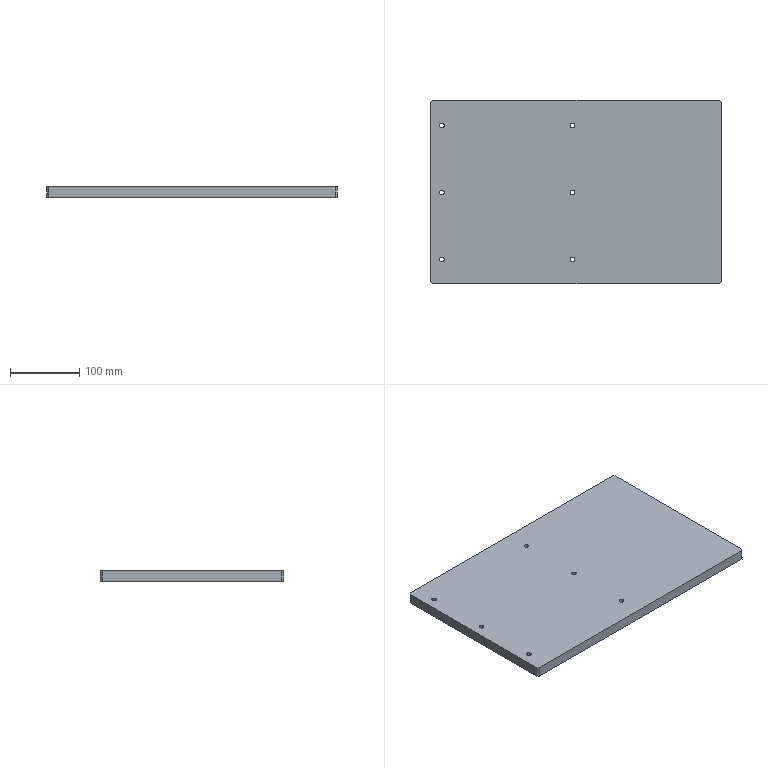Component | SolidWorks | STE21014.01-48-1 | 1 solid | 22 faces | box 420 x 265 x 15 mm | volume 1665961 mm3 | cylinder 12 | plane 10 | commonest cylinder face diameters 6.8 x12 | material Q235
build123d program:
from build123d import *

# Parameters (mm, degrees)
SKETCH1_W           = 420
SKETCH1_H           = 265
BOSS_EXTRUDE1_DEPTH = 15
M8_TAPPED_HOLE1_D   = 6.8
CHAMFER1_SIZE       = 3


with BuildPart() as part:
    # Sketch1 → Boss-Extrude1 (new body)
    with BuildSketch(Plane(origin=(0, 0, 0), x_dir=(1, 0, 0), z_dir=(0, 1, 0))):
        Rectangle(SKETCH1_W, SKETCH1_H)
    extrude(amount=BOSS_EXTRUDE1_DEPTH)

    # M8 Tapped Hole1 (through all)
    with Locations(Plane(origin=(0, 15, 0), x_dir=(1, 0, 0), z_dir=(0, 1, 0))):
        with Locations((5, -96.25), (194, -96.25), (5, 97.75), (194, 97.75), (5, 0.75), (194, 0.75)):
            Hole(M8_TAPPED_HOLE1_D / 2)

    # Chamfer1
    chamfer1_edges = [part.edges().sort_by_distance(p)[0] for p in [
        (-210, 7.5, -132.5),
        (210, 7.5, -132.5),
        (210, 7.5, 132.5),
        (-210, 7.5, 132.5),
    ]]
    chamfer(chamfer1_edges, length=CHAMFER1_SIZE)


solid = part.part

# Placed as in the assembly
solid = solid.moved(Location((530, 687.5, -105), (-90, 0, 180)))
STEP:
#1=COLOUR_RGB('',0.7922,0.8196,0.9333);
#2=FILL_AREA_STYLE_COLOUR('',#1);
#3=FILL_AREA_STYLE('',(#2));
#4=SURFACE_STYLE_FILL_AREA(#3);
#5=SURFACE_SIDE_STYLE('',(#4));
#6=SURFACE_STYLE_USAGE(.BOTH.,#5);
#7=PRESENTATION_STYLE_ASSIGNMENT((#6));
#8=CARTESIAN_POINT('',(20.669,30.722,-4.134));
#9=VERTEX_POINT('',#8);
#10=CARTESIAN_POINT('',(20.669,30.99,-4.134));
#11=VERTEX_POINT('',#10);
#12=CARTESIAN_POINT('',(20.669,30.856,-4.134));
#13=DIRECTION('',(0.,0.,1.));
#14=DIRECTION('',(0.,1.,0.));
#15=AXIS2_PLACEMENT_3D('',#12,#13,#14);
#16=CIRCLE('',#15,0.1339);
#17=EDGE_CURVE('',#9,#11,#16,.T.);
#18=ORIENTED_EDGE('',*,*,#17,.F.);
#19=CARTESIAN_POINT('',(20.669,30.722,-3.543));
#20=VERTEX_POINT('',#19);
#21=CARTESIAN_POINT('',(20.669,30.722,-3.543));
#22=DIRECTION('',(0.,0.,1.));
#23=VECTOR('',#22,39.37);
#24=LINE('',#21,#23);
#25=EDGE_CURVE('',#9,#20,#24,.T.);
#26=ORIENTED_EDGE('',*,*,#25,.T.);
#27=CARTESIAN_POINT('',(20.669,30.99,-3.543));
#28=VERTEX_POINT('',#27);
#29=CARTESIAN_POINT('',(20.669,30.856,-3.543));
#30=DIRECTION('',(0.,0.,1.));
#31=DIRECTION('',(0.,1.,0.));
#32=AXIS2_PLACEMENT_3D('',#29,#30,#31);
#33=CIRCLE('',#32,0.1339);
#34=EDGE_CURVE('',#20,#28,#33,.T.);
#35=ORIENTED_EDGE('',*,*,#34,.T.);
#36=CARTESIAN_POINT('',(20.669,30.99,-3.543));
#37=DIRECTION('',(0.,0.,1.));
#38=VECTOR('',#37,39.37);
#39=LINE('',#36,#38);
#40=EDGE_CURVE('',#11,#28,#39,.T.);
#41=ORIENTED_EDGE('',*,*,#40,.F.);
#42=EDGE_LOOP('',(#18,#26,#35,#41));
#43=FACE_OUTER_BOUND('',#42,.T.);
#44=CARTESIAN_POINT('',(20.669,30.856,-3.543));
#45=DIRECTION('',(0.,0.,1.));
#46=DIRECTION('',(0.,1.,0.));
#47=AXIS2_PLACEMENT_3D('',#44,#45,#46);
#48=CYLINDRICAL_SURFACE('',#47,0.1339);
#49=ADVANCED_FACE('',(#43),#48,.F.);
#50=CARTESIAN_POINT('',(13.228,30.722,-4.134));
#51=VERTEX_POINT('',#50);
#52=CARTESIAN_POINT('',(13.228,30.99,-4.134));
#53=VERTEX_POINT('',#52);
#54=CARTESIAN_POINT('',(13.228,30.856,-4.134));
#55=DIRECTION('',(0.,0.,1.));
#56=DIRECTION('',(0.,1.,0.));
#57=AXIS2_PLACEMENT_3D('',#54,#55,#56);
#58=CIRCLE('',#57,0.1339);
#59=EDGE_CURVE('',#51,#53,#58,.T.);
#60=ORIENTED_EDGE('',*,*,#59,.F.);
#61=CARTESIAN_POINT('',(13.228,30.722,-3.543));
#62=VERTEX_POINT('',#61);
#63=CARTESIAN_POINT('',(13.228,30.722,-3.543));
#64=DIRECTION('',(0.,0.,1.));
#65=VECTOR('',#64,39.37);
#66=LINE('',#63,#65);
#67=EDGE_CURVE('',#51,#62,#66,.T.);
#68=ORIENTED_EDGE('',*,*,#67,.T.);
#69=CARTESIAN_POINT('',(13.228,30.99,-3.543));
#70=VERTEX_POINT('',#69);
#71=CARTESIAN_POINT('',(13.228,30.856,-3.543));
#72=DIRECTION('',(0.,0.,1.));
#73=DIRECTION('',(0.,1.,0.));
#74=AXIS2_PLACEMENT_3D('',#71,#72,#73);
#75=CIRCLE('',#74,0.1339);
#76=EDGE_CURVE('',#62,#70,#75,.T.);
#77=ORIENTED_EDGE('',*,*,#76,.T.);
#78=CARTESIAN_POINT('',(13.228,30.99,-3.543));
#79=DIRECTION('',(0.,0.,1.));
#80=VECTOR('',#79,39.37);
#81=LINE('',#78,#80);
#82=EDGE_CURVE('',#53,#70,#81,.T.);
#83=ORIENTED_EDGE('',*,*,#82,.F.);
#84=EDGE_LOOP('',(#60,#68,#77,#83));
#85=FACE_OUTER_BOUND('',#84,.T.);
#86=CARTESIAN_POINT('',(13.228,30.856,-3.543));
#87=DIRECTION('',(0.,0.,1.));
#88=DIRECTION('',(0.,1.,0.));
#89=AXIS2_PLACEMENT_3D('',#86,#87,#88);
#90=CYLINDRICAL_SURFACE('',#89,0.1339);
#91=ADVANCED_FACE('',(#85),#90,.F.);
#92=CARTESIAN_POINT('',(20.669,23.085,-4.134));
#93=VERTEX_POINT('',#92);
#94=CARTESIAN_POINT('',(20.669,23.352,-4.134));
#95=VERTEX_POINT('',#94);
#96=CARTESIAN_POINT('',(20.669,23.219,-4.134));
#97=DIRECTION('',(0.,0.,1.));
#98=DIRECTION('',(0.,1.,0.));
#99=AXIS2_PLACEMENT_3D('',#96,#97,#98);
#100=CIRCLE('',#99,0.1339);
#101=EDGE_CURVE('',#93,#95,#100,.T.);
#102=ORIENTED_EDGE('',*,*,#101,.F.);
#103=CARTESIAN_POINT('',(20.669,23.085,-3.543));
#104=VERTEX_POINT('',#103);
#105=CARTESIAN_POINT('',(20.669,23.085,-3.543));
#106=DIRECTION('',(0.,0.,1.));
#107=VECTOR('',#106,39.37);
#108=LINE('',#105,#107);
#109=EDGE_CURVE('',#93,#104,#108,.T.);
#110=ORIENTED_EDGE('',*,*,#109,.T.);
#111=CARTESIAN_POINT('',(20.669,23.352,-3.543));
#112=VERTEX_POINT('',#111);
#113=CARTESIAN_POINT('',(20.669,23.219,-3.543));
#114=DIRECTION('',(0.,0.,1.));
#115=DIRECTION('',(0.,1.,0.));
#116=AXIS2_PLACEMENT_3D('',#113,#114,#115);
#117=CIRCLE('',#116,0.1339);
#118=EDGE_CURVE('',#104,#112,#117,.T.);
#119=ORIENTED_EDGE('',*,*,#118,.T.);
#120=CARTESIAN_POINT('',(20.669,23.352,-3.543));
#121=DIRECTION('',(0.,0.,1.));
#122=VECTOR('',#121,39.37);
#123=LINE('',#120,#122);
#124=EDGE_CURVE('',#95,#112,#123,.T.);
#125=ORIENTED_EDGE('',*,*,#124,.F.);
#126=EDGE_LOOP('',(#102,#110,#119,#125));
#127=FACE_OUTER_BOUND('',#126,.T.);
#128=CARTESIAN_POINT('',(20.669,23.219,-3.543));
#129=DIRECTION('',(0.,0.,1.));
#130=DIRECTION('',(0.,1.,0.));
#131=AXIS2_PLACEMENT_3D('',#128,#129,#130);
#132=CYLINDRICAL_SURFACE('',#131,0.1339);
#133=ADVANCED_FACE('',(#127),#132,.F.);
#134=CARTESIAN_POINT('',(13.228,23.085,-4.134));
#135=VERTEX_POINT('',#134);
#136=CARTESIAN_POINT('',(13.228,23.352,-4.134));
#137=VERTEX_POINT('',#136);
#138=CARTESIAN_POINT('',(13.228,23.219,-4.134));
#139=DIRECTION('',(0.,0.,1.));
#140=DIRECTION('',(0.,1.,0.));
#141=AXIS2_PLACEMENT_3D('',#138,#139,#140);
#142=CIRCLE('',#141,0.1339);
#143=EDGE_CURVE('',#135,#137,#142,.T.);
#144=ORIENTED_EDGE('',*,*,#143,.F.);
#145=CARTESIAN_POINT('',(13.228,23.085,-3.543));
#146=VERTEX_POINT('',#145);
#147=CARTESIAN_POINT('',(13.228,23.085,-3.543));
#148=DIRECTION('',(0.,0.,1.));
#149=VECTOR('',#148,39.37);
#150=LINE('',#147,#149);
#151=EDGE_CURVE('',#135,#146,#150,.T.);
#152=ORIENTED_EDGE('',*,*,#151,.T.);
#153=CARTESIAN_POINT('',(13.228,23.352,-3.543));
#154=VERTEX_POINT('',#153);
#155=CARTESIAN_POINT('',(13.228,23.219,-3.543));
#156=DIRECTION('',(0.,0.,1.));
#157=DIRECTION('',(0.,1.,0.));
#158=AXIS2_PLACEMENT_3D('',#155,#156,#157);
#159=CIRCLE('',#158,0.1339);
#160=EDGE_CURVE('',#146,#154,#159,.T.);
#161=ORIENTED_EDGE('',*,*,#160,.T.);
#162=CARTESIAN_POINT('',(13.228,23.352,-3.543));
#163=DIRECTION('',(0.,0.,1.));
#164=VECTOR('',#163,39.37);
#165=LINE('',#162,#164);
#166=EDGE_CURVE('',#137,#154,#165,.T.);
#167=ORIENTED_EDGE('',*,*,#166,.F.);
#168=EDGE_LOOP('',(#144,#152,#161,#167));
#169=FACE_OUTER_BOUND('',#168,.T.);
#170=CARTESIAN_POINT('',(13.228,23.219,-3.543));
#171=DIRECTION('',(0.,0.,1.));
#172=DIRECTION('',(0.,1.,0.));
#173=AXIS2_PLACEMENT_3D('',#170,#171,#172);
#174=CYLINDRICAL_SURFACE('',#173,0.1339);
#175=ADVANCED_FACE('',(#169),#174,.F.);
#176=CARTESIAN_POINT('',(20.669,26.904,-4.134));
#177=VERTEX_POINT('',#176);
#178=CARTESIAN_POINT('',(20.669,27.171,-4.134));
#179=VERTEX_POINT('',#178);
#180=CARTESIAN_POINT('',(20.669,27.037,-4.134));
#181=DIRECTION('',(0.,0.,1.));
#182=DIRECTION('',(0.,1.,0.));
#183=AXIS2_PLACEMENT_3D('',#180,#181,#182);
#184=CIRCLE('',#183,0.1339);
#185=EDGE_CURVE('',#177,#179,#184,.T.);
#186=ORIENTED_EDGE('',*,*,#185,.F.);
#187=CARTESIAN_POINT('',(20.669,26.904,-3.543));
#188=VERTEX_POINT('',#187);
#189=CARTESIAN_POINT('',(20.669,26.904,-3.543));
#190=DIRECTION('',(0.,0.,1.));
#191=VECTOR('',#190,39.37);
#192=LINE('',#189,#191);
#193=EDGE_CURVE('',#177,#188,#192,.T.);
#194=ORIENTED_EDGE('',*,*,#193,.T.);
#195=CARTESIAN_POINT('',(20.669,27.171,-3.543));
#196=VERTEX_POINT('',#195);
#197=CARTESIAN_POINT('',(20.669,27.037,-3.543));
#198=DIRECTION('',(0.,0.,1.));
#199=DIRECTION('',(0.,1.,0.));
#200=AXIS2_PLACEMENT_3D('',#197,#198,#199);
#201=CIRCLE('',#200,0.1339);
#202=EDGE_CURVE('',#188,#196,#201,.T.);
#203=ORIENTED_EDGE('',*,*,#202,.T.);
#204=CARTESIAN_POINT('',(20.669,27.171,-3.543));
#205=DIRECTION('',(0.,0.,1.));
#206=VECTOR('',#205,39.37);
#207=LINE('',#204,#206);
#208=EDGE_CURVE('',#179,#196,#207,.T.);
#209=ORIENTED_EDGE('',*,*,#208,.F.);
#210=EDGE_LOOP('',(#186,#194,#203,#209));
#211=FACE_OUTER_BOUND('',#210,.T.);
#212=CARTESIAN_POINT('',(20.669,27.037,-3.543));
#213=DIRECTION('',(0.,0.,1.));
#214=DIRECTION('',(0.,1.,0.));
#215=AXIS2_PLACEMENT_3D('',#212,#213,#214);
#216=CYLINDRICAL_SURFACE('',#215,0.1339);
#217=ADVANCED_FACE('',(#211),#216,.F.);
#218=CARTESIAN_POINT('',(13.228,26.904,-4.134));
#219=VERTEX_POINT('',#218);
#220=CARTESIAN_POINT('',(13.228,27.171,-4.134));
#221=VERTEX_POINT('',#220);
#222=CARTESIAN_POINT('',(13.228,27.037,-4.134));
#223=DIRECTION('',(0.,0.,1.));
#224=DIRECTION('',(0.,1.,0.));
#225=AXIS2_PLACEMENT_3D('',#222,#223,#224);
#226=CIRCLE('',#225,0.1339);
#227=EDGE_CURVE('',#219,#221,#226,.T.);
#228=ORIENTED_EDGE('',*,*,#227,.F.);
#229=CARTESIAN_POINT('',(13.228,26.904,-3.543));
#230=VERTEX_POINT('',#229);
#231=CARTESIAN_POINT('',(13.228,26.904,-3.543));
#232=DIRECTION('',(0.,0.,1.));
#233=VECTOR('',#232,39.37);
#234=LINE('',#231,#233);
#235=EDGE_CURVE('',#219,#230,#234,.T.);
#236=ORIENTED_EDGE('',*,*,#235,.T.);
#237=CARTESIAN_POINT('',(13.228,27.171,-3.543));
#238=VERTEX_POINT('',#237);
#239=CARTESIAN_POINT('',(13.228,27.037,-3.543));
#240=DIRECTION('',(0.,0.,1.));
#241=DIRECTION('',(0.,1.,0.));
#242=AXIS2_PLACEMENT_3D('',#239,#240,#241);
#243=CIRCLE('',#242,0.1339);
#244=EDGE_CURVE('',#230,#238,#243,.T.);
#245=ORIENTED_EDGE('',*,*,#244,.T.);
#246=CARTESIAN_POINT('',(13.228,27.171,-3.543));
#247=DIRECTION('',(0.,0.,1.));
#248=VECTOR('',#247,39.37);
#249=LINE('',#246,#248);
#250=EDGE_CURVE('',#221,#238,#249,.T.);
#251=ORIENTED_EDGE('',*,*,#250,.F.);
#252=EDGE_LOOP('',(#228,#236,#245,#251));
#253=FACE_OUTER_BOUND('',#252,.T.);
#254=CARTESIAN_POINT('',(13.228,27.037,-3.543));
#255=DIRECTION('',(0.,0.,1.));
#256=DIRECTION('',(0.,1.,0.));
#257=AXIS2_PLACEMENT_3D('',#254,#255,#256);
#258=CYLINDRICAL_SURFACE('',#257,0.1339);
#259=ADVANCED_FACE('',(#253),#258,.F.);
#260=CARTESIAN_POINT('',(29.134,21.969,-3.543));
#261=VERTEX_POINT('',#260);
#262=CARTESIAN_POINT('',(29.134,32.165,-3.543));
#263=VERTEX_POINT('',#262);
#264=CARTESIAN_POINT('',(29.134,32.283,-3.543));
#265=DIRECTION('',(0.,1.,-0.));
#266=VECTOR('',#265,39.37);
#267=LINE('',#264,#266);
#268=EDGE_CURVE('',#261,#263,#267,.T.);
#269=ORIENTED_EDGE('',*,*,#268,.F.);
#270=CARTESIAN_POINT('',(29.134,21.969,-4.134));
#271=VERTEX_POINT('',#270);
#272=CARTESIAN_POINT('',(29.134,21.969,-3.543));
#273=DIRECTION('',(-0.,-0.,-1.));
#274=VECTOR('',#273,39.37);
#275=LINE('',#272,#274);
#276=EDGE_CURVE('',#261,#271,#275,.T.);
#277=ORIENTED_EDGE('',*,*,#276,.T.);
#278=CARTESIAN_POINT('',(29.134,32.165,-4.134));
#279=VERTEX_POINT('',#278);
#280=CARTESIAN_POINT('',(29.134,32.283,-4.134));
#281=DIRECTION('',(0.,1.,-0.));
#282=VECTOR('',#281,39.37);
#283=LINE('',#280,#282);
#284=EDGE_CURVE('',#271,#279,#283,.T.);
#285=ORIENTED_EDGE('',*,*,#284,.T.);
#286=CARTESIAN_POINT('',(29.134,32.165,-3.543));
#287=DIRECTION('',(0.,0.,1.));
#288=VECTOR('',#287,39.37);
#289=LINE('',#286,#288);
#290=EDGE_CURVE('',#279,#263,#289,.T.);
#291=ORIENTED_EDGE('',*,*,#290,.T.);
#292=EDGE_LOOP('',(#269,#277,#285,#291));
#293=FACE_OUTER_BOUND('',#292,.T.);
#294=CARTESIAN_POINT('',(29.134,32.283,-3.543));
#295=DIRECTION('',(-1.,0.,0.));
#296=DIRECTION('',(-0.,-1.,0.));
#297=AXIS2_PLACEMENT_3D('',#294,#295,#296);
#298=PLANE('',#297);
#299=ADVANCED_FACE('',(#293),#298,.F.);
#300=CARTESIAN_POINT('',(29.016,32.283,-3.543));
#301=VERTEX_POINT('',#300);
#302=CARTESIAN_POINT('',(12.717,32.283,-3.543));
#303=VERTEX_POINT('',#302);
#304=CARTESIAN_POINT('',(12.598,32.283,-3.543));
#305=DIRECTION('',(-1.,-0.,0.));
#306=VECTOR('',#305,39.37);
#307=LINE('',#304,#306);
#308=EDGE_CURVE('',#301,#303,#307,.T.);
#309=ORIENTED_EDGE('',*,*,#308,.F.);
#310=CARTESIAN_POINT('',(29.016,32.283,-4.134));
#311=VERTEX_POINT('',#310);
#312=CARTESIAN_POINT('',(29.016,32.283,-3.543));
#313=DIRECTION('',(-0.,-0.,-1.));
#314=VECTOR('',#313,39.37);
#315=LINE('',#312,#314);
#316=EDGE_CURVE('',#301,#311,#315,.T.);
#317=ORIENTED_EDGE('',*,*,#316,.T.);
#318=CARTESIAN_POINT('',(12.717,32.283,-4.134));
#319=VERTEX_POINT('',#318);
#320=CARTESIAN_POINT('',(12.598,32.283,-4.134));
#321=DIRECTION('',(-1.,-0.,0.));
#322=VECTOR('',#321,39.37);
#323=LINE('',#320,#322);
#324=EDGE_CURVE('',#311,#319,#323,.T.);
#325=ORIENTED_EDGE('',*,*,#324,.T.);
#326=CARTESIAN_POINT('',(12.717,32.283,-3.543));
#327=DIRECTION('',(0.,0.,1.));
#328=VECTOR('',#327,39.37);
#329=LINE('',#326,#328);
#330=EDGE_CURVE('',#319,#303,#329,.T.);
#331=ORIENTED_EDGE('',*,*,#330,.T.);
#332=EDGE_LOOP('',(#309,#317,#325,#331));
#333=FACE_OUTER_BOUND('',#332,.T.);
#334=CARTESIAN_POINT('',(12.598,32.283,-3.543));
#335=DIRECTION('',(0.,-1.,0.));
#336=DIRECTION('',(1.,0.,-0.));
#337=AXIS2_PLACEMENT_3D('',#334,#335,#336);
#338=PLANE('',#337);
#339=ADVANCED_FACE('',(#333),#338,.F.);
#340=CARTESIAN_POINT('',(12.598,32.165,-3.543));
#341=VERTEX_POINT('',#340);
#342=CARTESIAN_POINT('',(12.598,21.969,-3.543));
#343=VERTEX_POINT('',#342);
#344=CARTESIAN_POINT('',(12.598,32.283,-3.543));
#345=DIRECTION('',(-0.,-1.,0.));
#346=VECTOR('',#345,39.37);
#347=LINE('',#344,#346);
#348=EDGE_CURVE('',#341,#343,#347,.T.);
#349=ORIENTED_EDGE('',*,*,#348,.F.);
#350=CARTESIAN_POINT('',(12.598,32.165,-4.134));
#351=VERTEX_POINT('',#350);
#352=CARTESIAN_POINT('',(12.598,32.165,-3.543));
#353=DIRECTION('',(-0.,-0.,-1.));
#354=VECTOR('',#353,39.37);
#355=LINE('',#352,#354);
#356=EDGE_CURVE('',#341,#351,#355,.T.);
#357=ORIENTED_EDGE('',*,*,#356,.T.);
#358=CARTESIAN_POINT('',(12.598,21.969,-4.134));
#359=VERTEX_POINT('',#358);
#360=CARTESIAN_POINT('',(12.598,32.283,-4.134));
#361=DIRECTION('',(-0.,-1.,0.));
#362=VECTOR('',#361,39.37);
#363=LINE('',#360,#362);
#364=EDGE_CURVE('',#351,#359,#363,.T.);
#365=ORIENTED_EDGE('',*,*,#364,.T.);
#366=CARTESIAN_POINT('',(12.598,21.969,-3.543));
#367=DIRECTION('',(0.,0.,1.));
#368=VECTOR('',#367,39.37);
#369=LINE('',#366,#368);
#370=EDGE_CURVE('',#359,#343,#369,.T.);
#371=ORIENTED_EDGE('',*,*,#370,.T.);
#372=EDGE_LOOP('',(#349,#357,#365,#371));
#373=FACE_OUTER_BOUND('',#372,.T.);
#374=CARTESIAN_POINT('',(12.598,32.283,-3.543));
#375=DIRECTION('',(1.,-0.,-0.));
#376=DIRECTION('',(0.,1.,-0.));
#377=AXIS2_PLACEMENT_3D('',#374,#375,#376);
#378=PLANE('',#377);
#379=ADVANCED_FACE('',(#373),#378,.F.);
#380=CARTESIAN_POINT('',(12.717,21.85,-4.134));
#381=VERTEX_POINT('',#380);
#382=CARTESIAN_POINT('',(29.016,21.85,-4.134));
#383=VERTEX_POINT('',#382);
#384=CARTESIAN_POINT('',(12.598,21.85,-4.134));
#385=DIRECTION('',(1.,0.,-0.));
#386=VECTOR('',#385,39.37);
#387=LINE('',#384,#386);
#388=EDGE_CURVE('',#381,#383,#387,.T.);
#389=ORIENTED_EDGE('',*,*,#388,.T.);
#390=CARTESIAN_POINT('',(29.016,21.85,-3.543));
#391=VERTEX_POINT('',#390);
#392=CARTESIAN_POINT('',(29.016,21.85,-3.543));
#393=DIRECTION('',(0.,0.,1.));
#394=VECTOR('',#393,39.37);
#395=LINE('',#392,#394);
#396=EDGE_CURVE('',#383,#391,#395,.T.);
#397=ORIENTED_EDGE('',*,*,#396,.T.);
#398=CARTESIAN_POINT('',(12.717,21.85,-3.543));
#399=VERTEX_POINT('',#398);
#400=CARTESIAN_POINT('',(12.598,21.85,-3.543));
#401=DIRECTION('',(1.,0.,-0.));
#402=VECTOR('',#401,39.37);
#403=LINE('',#400,#402);
#404=EDGE_CURVE('',#399,#391,#403,.T.);
#405=ORIENTED_EDGE('',*,*,#404,.F.);
#406=CARTESIAN_POINT('',(12.717,21.85,-3.543));
#407=DIRECTION('',(-0.,-0.,-1.));
#408=VECTOR('',#407,39.37);
#409=LINE('',#406,#408);
#410=EDGE_CURVE('',#399,#381,#409,.T.);
#411=ORIENTED_EDGE('',*,*,#410,.T.);
#412=EDGE_LOOP('',(#389,#397,#405,#411));
#413=FACE_OUTER_BOUND('',#412,.T.);
#414=CARTESIAN_POINT('',(12.598,21.85,-3.543));
#415=DIRECTION('',(-0.,1.,-0.));
#416=DIRECTION('',(-1.,-0.,0.));
#417=AXIS2_PLACEMENT_3D('',#414,#415,#416);
#418=PLANE('',#417);
#419=ADVANCED_FACE('',(#413),#418,.F.);
#420=CARTESIAN_POINT('',(20.669,30.856,-3.543));
#421=DIRECTION('',(0.,0.,1.));
#422=DIRECTION('',(0.,1.,0.));
#423=AXIS2_PLACEMENT_3D('',#420,#421,#422);
#424=CIRCLE('',#423,0.1339);
#425=EDGE_CURVE('',#28,#20,#424,.T.);
#426=ORIENTED_EDGE('',*,*,#425,.F.);
#427=ORIENTED_EDGE('',*,*,#34,.F.);
#428=EDGE_LOOP('',(#426,#427));
#429=FACE_BOUND('',#428,.T.);
#430=CARTESIAN_POINT('',(13.228,30.856,-3.543));
#431=DIRECTION('',(0.,0.,1.));
#432=DIRECTION('',(0.,1.,0.));
#433=AXIS2_PLACEMENT_3D('',#430,#431,#432);
#434=CIRCLE('',#433,0.1339);
#435=EDGE_CURVE('',#70,#62,#434,.T.);
#436=ORIENTED_EDGE('',*,*,#435,.F.);
#437=ORIENTED_EDGE('',*,*,#76,.F.);
#438=EDGE_LOOP('',(#436,#437));
#439=FACE_BOUND('',#438,.T.);
#440=CARTESIAN_POINT('',(20.669,23.219,-3.543));
#441=DIRECTION('',(0.,0.,1.));
#442=DIRECTION('',(0.,1.,0.));
#443=AXIS2_PLACEMENT_3D('',#440,#441,#442);
#444=CIRCLE('',#443,0.1339);
#445=EDGE_CURVE('',#112,#104,#444,.T.);
#446=ORIENTED_EDGE('',*,*,#445,.F.);
#447=ORIENTED_EDGE('',*,*,#118,.F.);
#448=EDGE_LOOP('',(#446,#447));
#449=FACE_BOUND('',#448,.T.);
#450=CARTESIAN_POINT('',(13.228,23.219,-3.543));
#451=DIRECTION('',(0.,0.,1.));
#452=DIRECTION('',(0.,1.,0.));
#453=AXIS2_PLACEMENT_3D('',#450,#451,#452);
#454=CIRCLE('',#453,0.1339);
#455=EDGE_CURVE('',#154,#146,#454,.T.);
#456=ORIENTED_EDGE('',*,*,#455,.F.);
#457=ORIENTED_EDGE('',*,*,#160,.F.);
#458=EDGE_LOOP('',(#456,#457));
#459=FACE_BOUND('',#458,.T.);
#460=CARTESIAN_POINT('',(20.669,27.037,-3.543));
#461=DIRECTION('',(0.,0.,1.));
#462=DIRECTION('',(0.,1.,0.));
#463=AXIS2_PLACEMENT_3D('',#460,#461,#462);
#464=CIRCLE('',#463,0.1339);
#465=EDGE_CURVE('',#196,#188,#464,.T.);
#466=ORIENTED_EDGE('',*,*,#465,.F.);
#467=ORIENTED_EDGE('',*,*,#202,.F.);
#468=EDGE_LOOP('',(#466,#467));
#469=FACE_BOUND('',#468,.T.);
#470=CARTESIAN_POINT('',(13.228,27.037,-3.543));
#471=DIRECTION('',(0.,0.,1.));
#472=DIRECTION('',(0.,1.,0.));
#473=AXIS2_PLACEMENT_3D('',#470,#471,#472);
#474=CIRCLE('',#473,0.1339);
#475=EDGE_CURVE('',#238,#230,#474,.T.);
#476=ORIENTED_EDGE('',*,*,#475,.F.);
#477=ORIENTED_EDGE('',*,*,#244,.F.);
#478=EDGE_LOOP('',(#476,#477));
#479=FACE_BOUND('',#478,.T.);
#480=ORIENTED_EDGE('',*,*,#404,.T.);
#481=CARTESIAN_POINT('',(27.549,20.384,-3.543));
#482=DIRECTION('',(0.7071,0.7071,-0.));
#483=VECTOR('',#482,39.37);
#484=LINE('',#481,#483);
#485=EDGE_CURVE('',#391,#261,#484,.T.);
#486=ORIENTED_EDGE('',*,*,#485,.T.);
#487=ORIENTED_EDGE('',*,*,#268,.T.);
#488=CARTESIAN_POINT('',(27.549,33.75,-3.543));
#489=DIRECTION('',(-0.7071,0.7071,0.));
#490=VECTOR('',#489,39.37);
#491=LINE('',#488,#490);
#492=EDGE_CURVE('',#263,#301,#491,.T.);
#493=ORIENTED_EDGE('',*,*,#492,.T.);
#494=ORIENTED_EDGE('',*,*,#308,.T.);
#495=CARTESIAN_POINT('',(14.183,33.75,-3.543));
#496=DIRECTION('',(-0.7071,-0.7071,0.));
#497=VECTOR('',#496,39.37);
#498=LINE('',#495,#497);
#499=EDGE_CURVE('',#303,#341,#498,.T.);
#500=ORIENTED_EDGE('',*,*,#499,.T.);
#501=ORIENTED_EDGE('',*,*,#348,.T.);
#502=CARTESIAN_POINT('',(14.183,20.384,-3.543));
#503=DIRECTION('',(0.7071,-0.7071,-0.));
#504=VECTOR('',#503,39.37);
#505=LINE('',#502,#504);
#506=EDGE_CURVE('',#343,#399,#505,.T.);
#507=ORIENTED_EDGE('',*,*,#506,.T.);
#508=EDGE_LOOP('',(#480,#486,#487,#493,#494,#500,#501,#507));
#509=FACE_OUTER_BOUND('',#508,.T.);
#510=CARTESIAN_POINT('',(20.866,27.067,-3.543));
#511=DIRECTION('',(0.,0.,1.));
#512=DIRECTION('',(0.,1.,-0.));
#513=AXIS2_PLACEMENT_3D('',#510,#511,#512);
#514=PLANE('',#513);
#515=ADVANCED_FACE('',(#429,#439,#449,#459,#469,#479,#509),#514,.T.);
#516=CARTESIAN_POINT('',(20.669,30.856,-4.134));
#517=DIRECTION('',(0.,0.,1.));
#518=DIRECTION('',(0.,1.,0.));
#519=AXIS2_PLACEMENT_3D('',#516,#517,#518);
#520=CIRCLE('',#519,0.1339);
#521=EDGE_CURVE('',#11,#9,#520,.T.);
#522=ORIENTED_EDGE('',*,*,#521,.T.);
#523=ORIENTED_EDGE('',*,*,#17,.T.);
#524=EDGE_LOOP('',(#522,#523));
#525=FACE_BOUND('',#524,.T.);
#526=CARTESIAN_POINT('',(13.228,30.856,-4.134));
#527=DIRECTION('',(0.,0.,1.));
#528=DIRECTION('',(0.,1.,0.));
#529=AXIS2_PLACEMENT_3D('',#526,#527,#528);
#530=CIRCLE('',#529,0.1339);
#531=EDGE_CURVE('',#53,#51,#530,.T.);
#532=ORIENTED_EDGE('',*,*,#531,.T.);
#533=ORIENTED_EDGE('',*,*,#59,.T.);
#534=EDGE_LOOP('',(#532,#533));
#535=FACE_BOUND('',#534,.T.);
#536=CARTESIAN_POINT('',(20.669,23.219,-4.134));
#537=DIRECTION('',(0.,0.,1.));
#538=DIRECTION('',(0.,1.,0.));
#539=AXIS2_PLACEMENT_3D('',#536,#537,#538);
#540=CIRCLE('',#539,0.1339);
#541=EDGE_CURVE('',#95,#93,#540,.T.);
#542=ORIENTED_EDGE('',*,*,#541,.T.);
#543=ORIENTED_EDGE('',*,*,#101,.T.);
#544=EDGE_LOOP('',(#542,#543));
#545=FACE_BOUND('',#544,.T.);
#546=CARTESIAN_POINT('',(13.228,23.219,-4.134));
#547=DIRECTION('',(0.,0.,1.));
#548=DIRECTION('',(0.,1.,0.));
#549=AXIS2_PLACEMENT_3D('',#546,#547,#548);
#550=CIRCLE('',#549,0.1339);
#551=EDGE_CURVE('',#137,#135,#550,.T.);
#552=ORIENTED_EDGE('',*,*,#551,.T.);
#553=ORIENTED_EDGE('',*,*,#143,.T.);
#554=EDGE_LOOP('',(#552,#553));
#555=FACE_BOUND('',#554,.T.);
#556=CARTESIAN_POINT('',(20.669,27.037,-4.134));
#557=DIRECTION('',(0.,0.,1.));
#558=DIRECTION('',(0.,1.,0.));
#559=AXIS2_PLACEMENT_3D('',#556,#557,#558);
#560=CIRCLE('',#559,0.1339);
#561=EDGE_CURVE('',#179,#177,#560,.T.);
#562=ORIENTED_EDGE('',*,*,#561,.T.);
#563=ORIENTED_EDGE('',*,*,#185,.T.);
#564=EDGE_LOOP('',(#562,#563));
#565=FACE_BOUND('',#564,.T.);
#566=CARTESIAN_POINT('',(13.228,27.037,-4.134));
#567=DIRECTION('',(0.,0.,1.));
#568=DIRECTION('',(0.,1.,0.));
#569=AXIS2_PLACEMENT_3D('',#566,#567,#568);
#570=CIRCLE('',#569,0.1339);
#571=EDGE_CURVE('',#221,#219,#570,.T.);
#572=ORIENTED_EDGE('',*,*,#571,.T.);
#573=ORIENTED_EDGE('',*,*,#227,.T.);
#574=EDGE_LOOP('',(#572,#573));
#575=FACE_BOUND('',#574,.T.);
#576=ORIENTED_EDGE('',*,*,#284,.F.);
#577=CARTESIAN_POINT('',(29.134,21.969,-4.134));
#578=DIRECTION('',(-0.7071,-0.7071,0.));
#579=VECTOR('',#578,39.37);
#580=LINE('',#577,#579);
#581=EDGE_CURVE('',#271,#383,#580,.T.);
#582=ORIENTED_EDGE('',*,*,#581,.T.);
#583=ORIENTED_EDGE('',*,*,#388,.F.);
#584=CARTESIAN_POINT('',(12.717,21.85,-4.134));
#585=DIRECTION('',(-0.7071,0.7071,0.));
#586=VECTOR('',#585,39.37);
#587=LINE('',#584,#586);
#588=EDGE_CURVE('',#381,#359,#587,.T.);
#589=ORIENTED_EDGE('',*,*,#588,.T.);
#590=ORIENTED_EDGE('',*,*,#364,.F.);
#591=CARTESIAN_POINT('',(12.598,32.165,-4.134));
#592=DIRECTION('',(0.7071,0.7071,-0.));
#593=VECTOR('',#592,39.37);
#594=LINE('',#591,#593);
#595=EDGE_CURVE('',#351,#319,#594,.T.);
#596=ORIENTED_EDGE('',*,*,#595,.T.);
#597=ORIENTED_EDGE('',*,*,#324,.F.);
#598=CARTESIAN_POINT('',(29.016,32.283,-4.134));
#599=DIRECTION('',(0.7071,-0.7071,-0.));
#600=VECTOR('',#599,39.37);
#601=LINE('',#598,#600);
#602=EDGE_CURVE('',#311,#279,#601,.T.);
#603=ORIENTED_EDGE('',*,*,#602,.T.);
#604=EDGE_LOOP('',(#576,#582,#583,#589,#590,#596,#597,#603));
#605=FACE_OUTER_BOUND('',#604,.T.);
#606=CARTESIAN_POINT('',(20.866,27.067,-4.134));
#607=DIRECTION('',(0.,0.,1.));
#608=DIRECTION('',(0.,1.,-0.));
#609=AXIS2_PLACEMENT_3D('',#606,#607,#608);
#610=PLANE('',#609);
#611=ADVANCED_FACE('',(#525,#535,#545,#555,#565,#575,#605),#610,.F.);
#612=ORIENTED_EDGE('',*,*,#235,.F.);
#613=ORIENTED_EDGE('',*,*,#571,.F.);
#614=ORIENTED_EDGE('',*,*,#250,.T.);
#615=ORIENTED_EDGE('',*,*,#475,.T.);
#616=EDGE_LOOP('',(#612,#613,#614,#615));
#617=FACE_OUTER_BOUND('',#616,.T.);
#618=CARTESIAN_POINT('',(13.228,27.037,-3.543));
#619=DIRECTION('',(0.,0.,1.));
#620=DIRECTION('',(0.,1.,0.));
#621=AXIS2_PLACEMENT_3D('',#618,#619,#620);
#622=CYLINDRICAL_SURFACE('',#621,0.1339);
#623=ADVANCED_FACE('',(#617),#622,.F.);
#624=ORIENTED_EDGE('',*,*,#193,.F.);
#625=ORIENTED_EDGE('',*,*,#561,.F.);
#626=ORIENTED_EDGE('',*,*,#208,.T.);
#627=ORIENTED_EDGE('',*,*,#465,.T.);
#628=EDGE_LOOP('',(#624,#625,#626,#627));
#629=FACE_OUTER_BOUND('',#628,.T.);
#630=CARTESIAN_POINT('',(20.669,27.037,-3.543));
#631=DIRECTION('',(0.,0.,1.));
#632=DIRECTION('',(0.,1.,0.));
#633=AXIS2_PLACEMENT_3D('',#630,#631,#632);
#634=CYLINDRICAL_SURFACE('',#633,0.1339);
#635=ADVANCED_FACE('',(#629),#634,.F.);
#636=ORIENTED_EDGE('',*,*,#151,.F.);
#637=ORIENTED_EDGE('',*,*,#551,.F.);
#638=ORIENTED_EDGE('',*,*,#166,.T.);
#639=ORIENTED_EDGE('',*,*,#455,.T.);
#640=EDGE_LOOP('',(#636,#637,#638,#639));
#641=FACE_OUTER_BOUND('',#640,.T.);
#642=CARTESIAN_POINT('',(13.228,23.219,-3.543));
#643=DIRECTION('',(0.,0.,1.));
#644=DIRECTION('',(0.,1.,0.));
#645=AXIS2_PLACEMENT_3D('',#642,#643,#644);
#646=CYLINDRICAL_SURFACE('',#645,0.1339);
#647=ADVANCED_FACE('',(#641),#646,.F.);
#648=ORIENTED_EDGE('',*,*,#109,.F.);
#649=ORIENTED_EDGE('',*,*,#541,.F.);
#650=ORIENTED_EDGE('',*,*,#124,.T.);
#651=ORIENTED_EDGE('',*,*,#445,.T.);
#652=EDGE_LOOP('',(#648,#649,#650,#651));
#653=FACE_OUTER_BOUND('',#652,.T.);
#654=CARTESIAN_POINT('',(20.669,23.219,-3.543));
#655=DIRECTION('',(0.,0.,1.));
#656=DIRECTION('',(0.,1.,0.));
#657=AXIS2_PLACEMENT_3D('',#654,#655,#656);
#658=CYLINDRICAL_SURFACE('',#657,0.1339);
#659=ADVANCED_FACE('',(#653),#658,.F.);
#660=ORIENTED_EDGE('',*,*,#67,.F.);
#661=ORIENTED_EDGE('',*,*,#531,.F.);
#662=ORIENTED_EDGE('',*,*,#82,.T.);
#663=ORIENTED_EDGE('',*,*,#435,.T.);
#664=EDGE_LOOP('',(#660,#661,#662,#663));
#665=FACE_OUTER_BOUND('',#664,.T.);
#666=CARTESIAN_POINT('',(13.228,30.856,-3.543));
#667=DIRECTION('',(0.,0.,1.));
#668=DIRECTION('',(0.,1.,0.));
#669=AXIS2_PLACEMENT_3D('',#666,#667,#668);
#670=CYLINDRICAL_SURFACE('',#669,0.1339);
#671=ADVANCED_FACE('',(#665),#670,.F.);
#672=ORIENTED_EDGE('',*,*,#25,.F.);
#673=ORIENTED_EDGE('',*,*,#521,.F.);
#674=ORIENTED_EDGE('',*,*,#40,.T.);
#675=ORIENTED_EDGE('',*,*,#425,.T.);
#676=EDGE_LOOP('',(#672,#673,#674,#675));
#677=FACE_OUTER_BOUND('',#676,.T.);
#678=CARTESIAN_POINT('',(20.669,30.856,-3.543));
#679=DIRECTION('',(0.,0.,1.));
#680=DIRECTION('',(0.,1.,0.));
#681=AXIS2_PLACEMENT_3D('',#678,#679,#680);
#682=CYLINDRICAL_SURFACE('',#681,0.1339);
#683=ADVANCED_FACE('',(#677),#682,.F.);
#684=ORIENTED_EDGE('',*,*,#485,.F.);
#685=ORIENTED_EDGE('',*,*,#396,.F.);
#686=ORIENTED_EDGE('',*,*,#581,.F.);
#687=ORIENTED_EDGE('',*,*,#276,.F.);
#688=EDGE_LOOP('',(#684,#685,#686,#687));
#689=FACE_OUTER_BOUND('',#688,.T.);
#690=CARTESIAN_POINT('',(29.134,21.969,-3.543));
#691=DIRECTION('',(-0.7071,0.7071,0.));
#692=DIRECTION('',(-0.,-0.,-1.));
#693=AXIS2_PLACEMENT_3D('',#690,#691,#692);
#694=PLANE('',#693);
#695=ADVANCED_FACE('',(#689),#694,.F.);
#696=ORIENTED_EDGE('',*,*,#492,.F.);
#697=ORIENTED_EDGE('',*,*,#290,.F.);
#698=ORIENTED_EDGE('',*,*,#602,.F.);
#699=ORIENTED_EDGE('',*,*,#316,.F.);
#700=EDGE_LOOP('',(#696,#697,#698,#699));
#701=FACE_OUTER_BOUND('',#700,.T.);
#702=CARTESIAN_POINT('',(29.016,32.283,-3.543));
#703=DIRECTION('',(-0.7071,-0.7071,0.));
#704=DIRECTION('',(-0.,-0.,-1.));
#705=AXIS2_PLACEMENT_3D('',#702,#703,#704);
#706=PLANE('',#705);
#707=ADVANCED_FACE('',(#701),#706,.F.);
#708=ORIENTED_EDGE('',*,*,#499,.F.);
#709=ORIENTED_EDGE('',*,*,#330,.F.);
#710=ORIENTED_EDGE('',*,*,#595,.F.);
#711=ORIENTED_EDGE('',*,*,#356,.F.);
#712=EDGE_LOOP('',(#708,#709,#710,#711));
#713=FACE_OUTER_BOUND('',#712,.T.);
#714=CARTESIAN_POINT('',(12.598,32.165,-3.543));
#715=DIRECTION('',(0.7071,-0.7071,-0.));
#716=DIRECTION('',(-0.,-0.,-1.));
#717=AXIS2_PLACEMENT_3D('',#714,#715,#716);
#718=PLANE('',#717);
#719=ADVANCED_FACE('',(#713),#718,.F.);
#720=ORIENTED_EDGE('',*,*,#506,.F.);
#721=ORIENTED_EDGE('',*,*,#370,.F.);
#722=ORIENTED_EDGE('',*,*,#588,.F.);
#723=ORIENTED_EDGE('',*,*,#410,.F.);
#724=EDGE_LOOP('',(#720,#721,#722,#723));
#725=FACE_OUTER_BOUND('',#724,.T.);
#726=CARTESIAN_POINT('',(12.717,21.85,-3.543));
#727=DIRECTION('',(0.7071,0.7071,-0.));
#728=DIRECTION('',(-0.,-0.,-1.));
#729=AXIS2_PLACEMENT_3D('',#726,#727,#728);
#730=PLANE('',#729);
#731=ADVANCED_FACE('',(#725),#730,.F.);
#732=CLOSED_SHELL('',(#49,#91,#133,#175,#217,#259,#299,#339,#379,#419,#515,#611,#623,#635,#647,#659,#671,#683,#695,#707,#719,#731));
#733=MANIFOLD_SOLID_BREP('',#732);
#734=STYLED_ITEM('',(#7),#733);
#735=PRESENTATION_LAYER_ASSIGNMENT('','',(#734));
#736=CARTESIAN_POINT('',(0.,0.,0.));
#737=DIRECTION('',(0.,0.,1.));
#738=DIRECTION('',(1.,0.,0.));
#739=AXIS2_PLACEMENT_3D('',#736,#737,#738);
#740=(LENGTH_UNIT()NAMED_UNIT(*)SI_UNIT($,.METRE.));
#741=LENGTH_MEASURE_WITH_UNIT(LENGTH_MEASURE(0.0254),#740);
#742=DIMENSIONAL_EXPONENTS(1.,0.,0.,0.,0.,0.,0.);
#743=(CONVERSION_BASED_UNIT('',#741)LENGTH_UNIT()NAMED_UNIT(#742));
#744=UNCERTAINTY_MEASURE_WITH_UNIT(LENGTH_MEASURE(0.00001),#743,'','');
#745=(NAMED_UNIT(*)PLANE_ANGLE_UNIT()SI_UNIT($,.RADIAN.));
#746=(NAMED_UNIT(*)SI_UNIT($,.STERADIAN.)SOLID_ANGLE_UNIT());
#747=(GEOMETRIC_REPRESENTATION_CONTEXT(3)GLOBAL_UNCERTAINTY_ASSIGNED_CONTEXT((#744))GLOBAL_UNIT_ASSIGNED_CONTEXT((#743,#745,#746))REPRESENTATION_CONTEXT('',''));
#748=ADVANCED_BREP_SHAPE_REPRESENTATION('',(#733,#739),#747);
#749=(LENGTH_UNIT()NAMED_UNIT(*)SI_UNIT($,.METRE.));
#750=LENGTH_MEASURE_WITH_UNIT(LENGTH_MEASURE(0.0254),#749);
#751=DIMENSIONAL_EXPONENTS(1.,0.,0.,0.,0.,0.,0.);
#752=(CONVERSION_BASED_UNIT('',#750)LENGTH_UNIT()NAMED_UNIT(#751));
#753=UNCERTAINTY_MEASURE_WITH_UNIT(LENGTH_MEASURE(0.00001),#752,'','');
#754=(NAMED_UNIT(*)PLANE_ANGLE_UNIT()SI_UNIT($,.RADIAN.));
#755=(NAMED_UNIT(*)SI_UNIT($,.STERADIAN.)SOLID_ANGLE_UNIT());
#756=(GEOMETRIC_REPRESENTATION_CONTEXT(3)GLOBAL_UNCERTAINTY_ASSIGNED_CONTEXT((#753))GLOBAL_UNIT_ASSIGNED_CONTEXT((#752,#754,#755))REPRESENTATION_CONTEXT('',''));
#757=MECHANICAL_DESIGN_GEOMETRIC_PRESENTATION_REPRESENTATION('',(#734),#756);